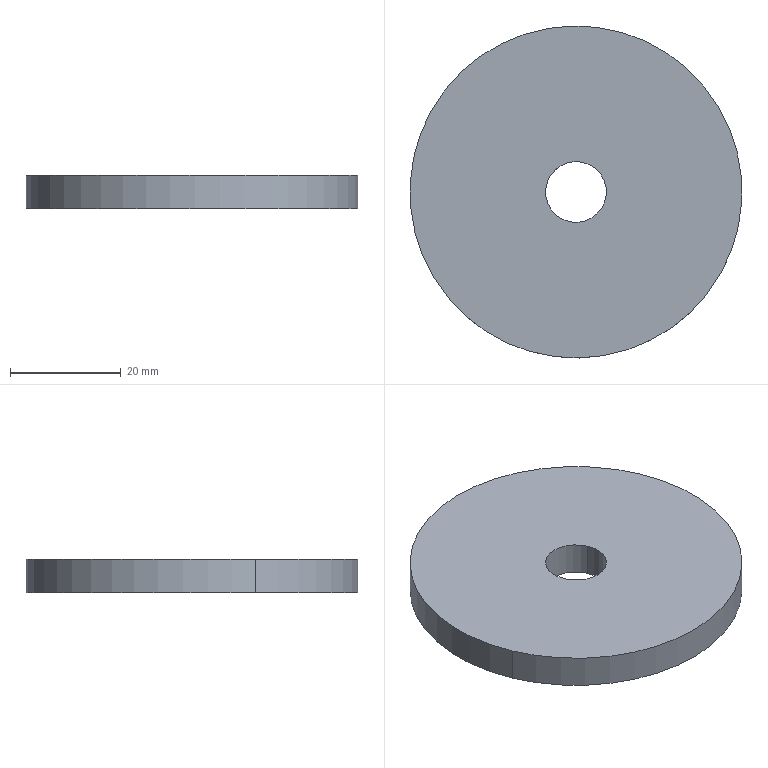Component | SolidWorks | 12AFixedLargeStraighteningWheelBaffle-12 | 1 solid | 6 faces | box 60 x 60 x 6 mm | volume 16394 mm3 | cylinder 4 | plane 2 | commonest cylinder face diameters 11 x2 60 x2 | material Q235
build123d program:
from build123d import *

# Parameters (mm, degrees)
SKETCH1_R           = 30
SKETCH1_R_2         = 5.5
BOSS_EXTRUDE1_DEPTH = 6


with BuildPart() as part:
    # Sketch1 → Boss-Extrude1 (new body)
    with BuildSketch(Plane.XY):
        Circle(SKETCH1_R)
        Circle(SKETCH1_R_2, mode=Mode.SUBTRACT)
    extrude(amount=BOSS_EXTRUDE1_DEPTH)


solid = part.part

# Placed as in the assembly
solid = solid.moved(Location((-349.402, 59.038, -20.25), (0, 0, 0)))
STEP:
#1=COLOUR_RGB('',0.7922,0.8196,0.9333);
#2=FILL_AREA_STYLE_COLOUR('',#1);
#3=FILL_AREA_STYLE('',(#2));
#4=SURFACE_STYLE_FILL_AREA(#3);
#5=SURFACE_SIDE_STYLE('',(#4));
#6=SURFACE_STYLE_USAGE(.BOTH.,#5);
#7=PRESENTATION_STYLE_ASSIGNMENT((#6));
#8=CARTESIAN_POINT('',(-13.556,2.407,-0.7972));
#9=VERTEX_POINT('',#8);
#10=CARTESIAN_POINT('',(-13.956,2.241,-0.7972));
#11=VERTEX_POINT('',#10);
#12=CARTESIAN_POINT('',(-13.756,2.324,-0.7972));
#13=DIRECTION('',(0.,0.,-1.));
#14=DIRECTION('',(-0.9237,-0.383,0.));
#15=AXIS2_PLACEMENT_3D('',#12,#13,#14);
#16=CIRCLE('',#15,0.2165);
#17=EDGE_CURVE('',#9,#11,#16,.T.);
#18=ORIENTED_EDGE('',*,*,#17,.T.);
#19=CARTESIAN_POINT('',(-13.956,2.241,-0.561));
#20=VERTEX_POINT('',#19);
#21=CARTESIAN_POINT('',(-13.956,2.241,-0.7972));
#22=DIRECTION('',(0.,0.,1.));
#23=VECTOR('',#22,39.37);
#24=LINE('',#21,#23);
#25=EDGE_CURVE('',#11,#20,#24,.T.);
#26=ORIENTED_EDGE('',*,*,#25,.T.);
#27=CARTESIAN_POINT('',(-13.556,2.407,-0.561));
#28=VERTEX_POINT('',#27);
#29=CARTESIAN_POINT('',(-13.756,2.324,-0.561));
#30=DIRECTION('',(0.,0.,-1.));
#31=DIRECTION('',(-0.9237,-0.383,0.));
#32=AXIS2_PLACEMENT_3D('',#29,#30,#31);
#33=CIRCLE('',#32,0.2165);
#34=EDGE_CURVE('',#28,#20,#33,.T.);
#35=ORIENTED_EDGE('',*,*,#34,.F.);
#36=CARTESIAN_POINT('',(-13.556,2.407,-0.7972));
#37=DIRECTION('',(0.,0.,1.));
#38=VECTOR('',#37,39.37);
#39=LINE('',#36,#38);
#40=EDGE_CURVE('',#9,#28,#39,.T.);
#41=ORIENTED_EDGE('',*,*,#40,.F.);
#42=EDGE_LOOP('',(#18,#26,#35,#41));
#43=FACE_OUTER_BOUND('',#42,.T.);
#44=CARTESIAN_POINT('',(-13.756,2.324,-0.7972));
#45=DIRECTION('',(0.,0.,1.));
#46=DIRECTION('',(0.9237,0.383,0.));
#47=AXIS2_PLACEMENT_3D('',#44,#45,#46);
#48=CYLINDRICAL_SURFACE('',#47,0.2165);
#49=ADVANCED_FACE('',(#43),#48,.F.);
#50=CARTESIAN_POINT('',(-14.847,1.872,-0.7972));
#51=VERTEX_POINT('',#50);
#52=CARTESIAN_POINT('',(-12.665,2.777,-0.7972));
#53=VERTEX_POINT('',#52);
#54=CARTESIAN_POINT('',(-13.756,2.324,-0.7972));
#55=DIRECTION('',(0.,0.,-1.));
#56=DIRECTION('',(-0.9237,-0.383,0.));
#57=AXIS2_PLACEMENT_3D('',#54,#55,#56);
#58=CIRCLE('',#57,1.181);
#59=EDGE_CURVE('',#51,#53,#58,.T.);
#60=ORIENTED_EDGE('',*,*,#59,.F.);
#61=CARTESIAN_POINT('',(-14.847,1.872,-0.561));
#62=VERTEX_POINT('',#61);
#63=CARTESIAN_POINT('',(-14.847,1.872,-0.7972));
#64=DIRECTION('',(0.,0.,1.));
#65=VECTOR('',#64,39.37);
#66=LINE('',#63,#65);
#67=EDGE_CURVE('',#51,#62,#66,.T.);
#68=ORIENTED_EDGE('',*,*,#67,.T.);
#69=CARTESIAN_POINT('',(-12.665,2.777,-0.561));
#70=VERTEX_POINT('',#69);
#71=CARTESIAN_POINT('',(-13.756,2.324,-0.561));
#72=DIRECTION('',(0.,0.,-1.));
#73=DIRECTION('',(-0.9237,-0.383,0.));
#74=AXIS2_PLACEMENT_3D('',#71,#72,#73);
#75=CIRCLE('',#74,1.181);
#76=EDGE_CURVE('',#62,#70,#75,.T.);
#77=ORIENTED_EDGE('',*,*,#76,.T.);
#78=CARTESIAN_POINT('',(-12.665,2.777,-0.7972));
#79=DIRECTION('',(0.,0.,1.));
#80=VECTOR('',#79,39.37);
#81=LINE('',#78,#80);
#82=EDGE_CURVE('',#53,#70,#81,.T.);
#83=ORIENTED_EDGE('',*,*,#82,.F.);
#84=EDGE_LOOP('',(#60,#68,#77,#83));
#85=FACE_OUTER_BOUND('',#84,.T.);
#86=CARTESIAN_POINT('',(-13.756,2.324,-0.7972));
#87=DIRECTION('',(0.,0.,1.));
#88=DIRECTION('',(0.9237,0.383,0.));
#89=AXIS2_PLACEMENT_3D('',#86,#87,#88);
#90=CYLINDRICAL_SURFACE('',#89,1.181);
#91=ADVANCED_FACE('',(#85),#90,.T.);
#92=CARTESIAN_POINT('',(-13.756,2.324,-0.7972));
#93=DIRECTION('',(0.,0.,-1.));
#94=DIRECTION('',(-0.9237,-0.383,0.));
#95=AXIS2_PLACEMENT_3D('',#92,#93,#94);
#96=CIRCLE('',#95,1.181);
#97=EDGE_CURVE('',#53,#51,#96,.T.);
#98=ORIENTED_EDGE('',*,*,#97,.T.);
#99=ORIENTED_EDGE('',*,*,#59,.T.);
#100=EDGE_LOOP('',(#98,#99));
#101=FACE_OUTER_BOUND('',#100,.T.);
#102=ORIENTED_EDGE('',*,*,#17,.F.);
#103=CARTESIAN_POINT('',(-13.756,2.324,-0.7972));
#104=DIRECTION('',(0.,0.,-1.));
#105=DIRECTION('',(-0.9237,-0.383,0.));
#106=AXIS2_PLACEMENT_3D('',#103,#104,#105);
#107=CIRCLE('',#106,0.2165);
#108=EDGE_CURVE('',#11,#9,#107,.T.);
#109=ORIENTED_EDGE('',*,*,#108,.F.);
#110=EDGE_LOOP('',(#102,#109));
#111=FACE_BOUND('',#110,.T.);
#112=CARTESIAN_POINT('',(-13.756,2.324,-0.7972));
#113=DIRECTION('',(0.,0.,-1.));
#114=DIRECTION('',(-0.9237,-0.383,0.));
#115=AXIS2_PLACEMENT_3D('',#112,#113,#114);
#116=PLANE('',#115);
#117=ADVANCED_FACE('',(#101,#111),#116,.T.);
#118=CARTESIAN_POINT('',(-13.756,2.324,-0.561));
#119=DIRECTION('',(0.,0.,-1.));
#120=DIRECTION('',(-0.9237,-0.383,0.));
#121=AXIS2_PLACEMENT_3D('',#118,#119,#120);
#122=CIRCLE('',#121,1.181);
#123=EDGE_CURVE('',#70,#62,#122,.T.);
#124=ORIENTED_EDGE('',*,*,#123,.F.);
#125=ORIENTED_EDGE('',*,*,#76,.F.);
#126=EDGE_LOOP('',(#124,#125));
#127=FACE_OUTER_BOUND('',#126,.T.);
#128=ORIENTED_EDGE('',*,*,#34,.T.);
#129=CARTESIAN_POINT('',(-13.756,2.324,-0.561));
#130=DIRECTION('',(0.,0.,-1.));
#131=DIRECTION('',(-0.9237,-0.383,0.));
#132=AXIS2_PLACEMENT_3D('',#129,#130,#131);
#133=CIRCLE('',#132,0.2165);
#134=EDGE_CURVE('',#20,#28,#133,.T.);
#135=ORIENTED_EDGE('',*,*,#134,.T.);
#136=EDGE_LOOP('',(#128,#135));
#137=FACE_BOUND('',#136,.T.);
#138=CARTESIAN_POINT('',(-13.756,2.324,-0.561));
#139=DIRECTION('',(0.,0.,-1.));
#140=DIRECTION('',(-0.9237,-0.383,0.));
#141=AXIS2_PLACEMENT_3D('',#138,#139,#140);
#142=PLANE('',#141);
#143=ADVANCED_FACE('',(#127,#137),#142,.F.);
#144=ORIENTED_EDGE('',*,*,#67,.F.);
#145=ORIENTED_EDGE('',*,*,#97,.F.);
#146=ORIENTED_EDGE('',*,*,#82,.T.);
#147=ORIENTED_EDGE('',*,*,#123,.T.);
#148=EDGE_LOOP('',(#144,#145,#146,#147));
#149=FACE_OUTER_BOUND('',#148,.T.);
#150=CARTESIAN_POINT('',(-13.756,2.324,-0.7972));
#151=DIRECTION('',(0.,0.,1.));
#152=DIRECTION('',(0.9237,0.383,0.));
#153=AXIS2_PLACEMENT_3D('',#150,#151,#152);
#154=CYLINDRICAL_SURFACE('',#153,1.181);
#155=ADVANCED_FACE('',(#149),#154,.T.);
#156=ORIENTED_EDGE('',*,*,#25,.F.);
#157=ORIENTED_EDGE('',*,*,#108,.T.);
#158=ORIENTED_EDGE('',*,*,#40,.T.);
#159=ORIENTED_EDGE('',*,*,#134,.F.);
#160=EDGE_LOOP('',(#156,#157,#158,#159));
#161=FACE_OUTER_BOUND('',#160,.T.);
#162=CARTESIAN_POINT('',(-13.756,2.324,-0.7972));
#163=DIRECTION('',(0.,0.,1.));
#164=DIRECTION('',(0.9237,0.383,0.));
#165=AXIS2_PLACEMENT_3D('',#162,#163,#164);
#166=CYLINDRICAL_SURFACE('',#165,0.2165);
#167=ADVANCED_FACE('',(#161),#166,.F.);
#168=CLOSED_SHELL('',(#49,#91,#117,#143,#155,#167));
#169=MANIFOLD_SOLID_BREP('',#168);
#170=STYLED_ITEM('',(#7),#169);
#171=(LENGTH_UNIT()NAMED_UNIT(*)SI_UNIT($,.METRE.));
#172=LENGTH_MEASURE_WITH_UNIT(LENGTH_MEASURE(0.0254),#171);
#173=DIMENSIONAL_EXPONENTS(1.,0.,0.,0.,0.,0.,0.);
#174=(CONVERSION_BASED_UNIT('',#172)LENGTH_UNIT()NAMED_UNIT(#173));
#175=UNCERTAINTY_MEASURE_WITH_UNIT(LENGTH_MEASURE(0.00001),#174,'','');
#176=(NAMED_UNIT(*)PLANE_ANGLE_UNIT()SI_UNIT($,.RADIAN.));
#177=(NAMED_UNIT(*)SI_UNIT($,.STERADIAN.)SOLID_ANGLE_UNIT());
#178=(GEOMETRIC_REPRESENTATION_CONTEXT(3)GLOBAL_UNCERTAINTY_ASSIGNED_CONTEXT((#175))GLOBAL_UNIT_ASSIGNED_CONTEXT((#174,#176,#177))REPRESENTATION_CONTEXT('',''));
#179=MECHANICAL_DESIGN_GEOMETRIC_PRESENTATION_REPRESENTATION('',(#170),#178);
#180=PRESENTATION_LAYER_ASSIGNMENT('','',(#170));
#181=CARTESIAN_POINT('',(0.,0.,0.));
#182=DIRECTION('',(0.,0.,1.));
#183=DIRECTION('',(1.,0.,0.));
#184=AXIS2_PLACEMENT_3D('',#181,#182,#183);
#185=(LENGTH_UNIT()NAMED_UNIT(*)SI_UNIT($,.METRE.));
#186=LENGTH_MEASURE_WITH_UNIT(LENGTH_MEASURE(0.0254),#185);
#187=DIMENSIONAL_EXPONENTS(1.,0.,0.,0.,0.,0.,0.);
#188=(CONVERSION_BASED_UNIT('',#186)LENGTH_UNIT()NAMED_UNIT(#187));
#189=UNCERTAINTY_MEASURE_WITH_UNIT(LENGTH_MEASURE(0.00001),#188,'','');
#190=(NAMED_UNIT(*)PLANE_ANGLE_UNIT()SI_UNIT($,.RADIAN.));
#191=(NAMED_UNIT(*)SI_UNIT($,.STERADIAN.)SOLID_ANGLE_UNIT());
#192=(GEOMETRIC_REPRESENTATION_CONTEXT(3)GLOBAL_UNCERTAINTY_ASSIGNED_CONTEXT((#189))GLOBAL_UNIT_ASSIGNED_CONTEXT((#188,#190,#191))REPRESENTATION_CONTEXT('',''));
#193=ADVANCED_BREP_SHAPE_REPRESENTATION('',(#169,#184),#192);